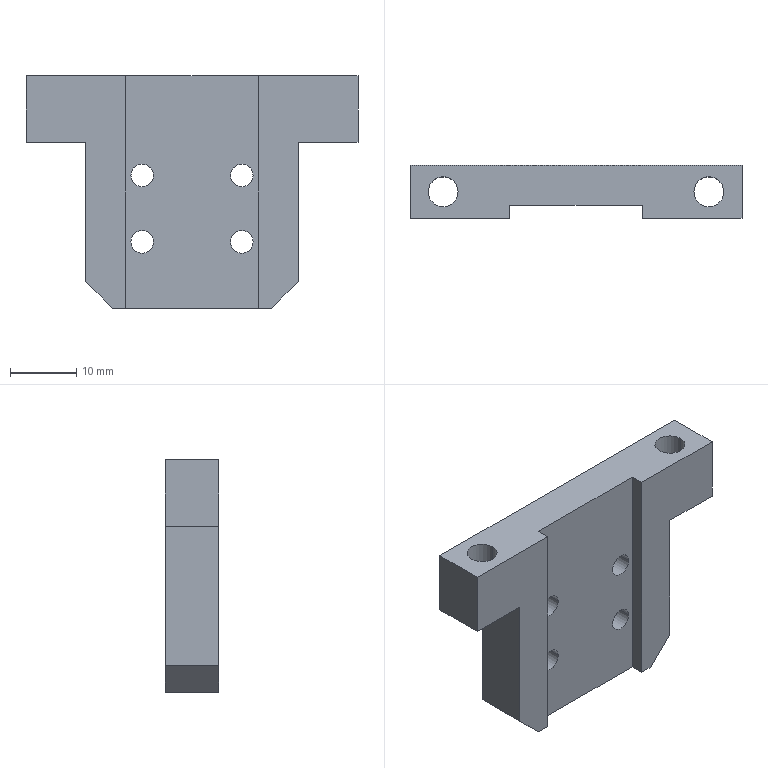Component | SolidWorks | P-SLJ-002-2_P-SLJ-002-002-1 | 1 solid | 40 faces | box 50 x 8 x 35 mm | volume 8075 mm3 | cylinder 20 | plane 20 | commonest cylinder face diameters 6 x8 3.4 x8 4.5 x4 | material Al 6061
build123d program:
from build123d import *

# Parameters (mm, degrees)
EXTRUDE1_DEPTH                                       = 4
SKETCH2_W                                            = 20
SKETCH2_H                                            = 2
EXTRUDE2_DEPTH                                       = 44.197
CBORE_FOR_M3_HEXAGON_SOCKET_HEAD_CAP_SCR_D           = 3.4
CBORE_FOR_M3_HEXAGON_SOCKET_HEAD_CAP_SCR_CBORE_D     = 6
CBORE_FOR_M3_HEXAGON_SOCKET_HEAD_CAP_SCR_CBORE_DEPTH = 3.4
M4_CLEARANCE_HOLE1_D                                 = 4.5
CHAMFER1_SIZE                                        = 4


with BuildPart() as part:
    # Sketch1 → Extrude1 (new, symmetric)
    with BuildSketch(Plane(origin=(0, 0, 0), x_dir=(1, 0, 0), z_dir=(0, 1, 0))):
        Polygon((5, 16), (5, 25), (-5, 25), (-5, -25), (5, -25), (5, -16), (30, -16), (30, 16), align=None)
    extrude(amount=EXTRUDE1_DEPTH, both=True)

    # Sketch2 → Extrude2 (cut, through all)
    with BuildSketch(Plane(origin=(30, 0, 0), x_dir=(0, 0, -1), z_dir=(1, 0, 0))):
        with Locations((0, -3)):
            Rectangle(SKETCH2_W, SKETCH2_H)
    extrude(amount=-EXTRUDE2_DEPTH, mode=Mode.SUBTRACT)

    # CBORE for M3 Hexagon socket head cap scr (through all)
    with Locations(Plane(origin=(0, 4, 0), x_dir=(1, 0, 0), z_dir=(0, 1, 0))):
        with Locations((10, 7.5), (10, -7.5), (20, 7.5), (20, -7.5)):
            CounterBoreHole(CBORE_FOR_M3_HEXAGON_SOCKET_HEAD_CAP_SCR_D / 2, CBORE_FOR_M3_HEXAGON_SOCKET_HEAD_CAP_SCR_CBORE_D / 2, CBORE_FOR_M3_HEXAGON_SOCKET_HEAD_CAP_SCR_CBORE_DEPTH)

    # M4 Clearance Hole1 (through all)
    with Locations(Plane(origin=(5, 0, 0), x_dir=(0, 0, -1), z_dir=(1, 0, 0))):
        with Locations((-20, 0), (20, 0)):
            Hole(M4_CLEARANCE_HOLE1_D / 2)

    # Chamfer1
    chamfer1_edges = [part.edges().sort_by_distance(p)[0] for p in [
        (30, 0, -16),
        (30, 0, 16),
    ]]
    chamfer(chamfer1_edges, length=CHAMFER1_SIZE)


solid = part.part

# Placed as in the assembly
solid = solid.moved(Location((-245, -61, 923.634), (0, 90, 0)))